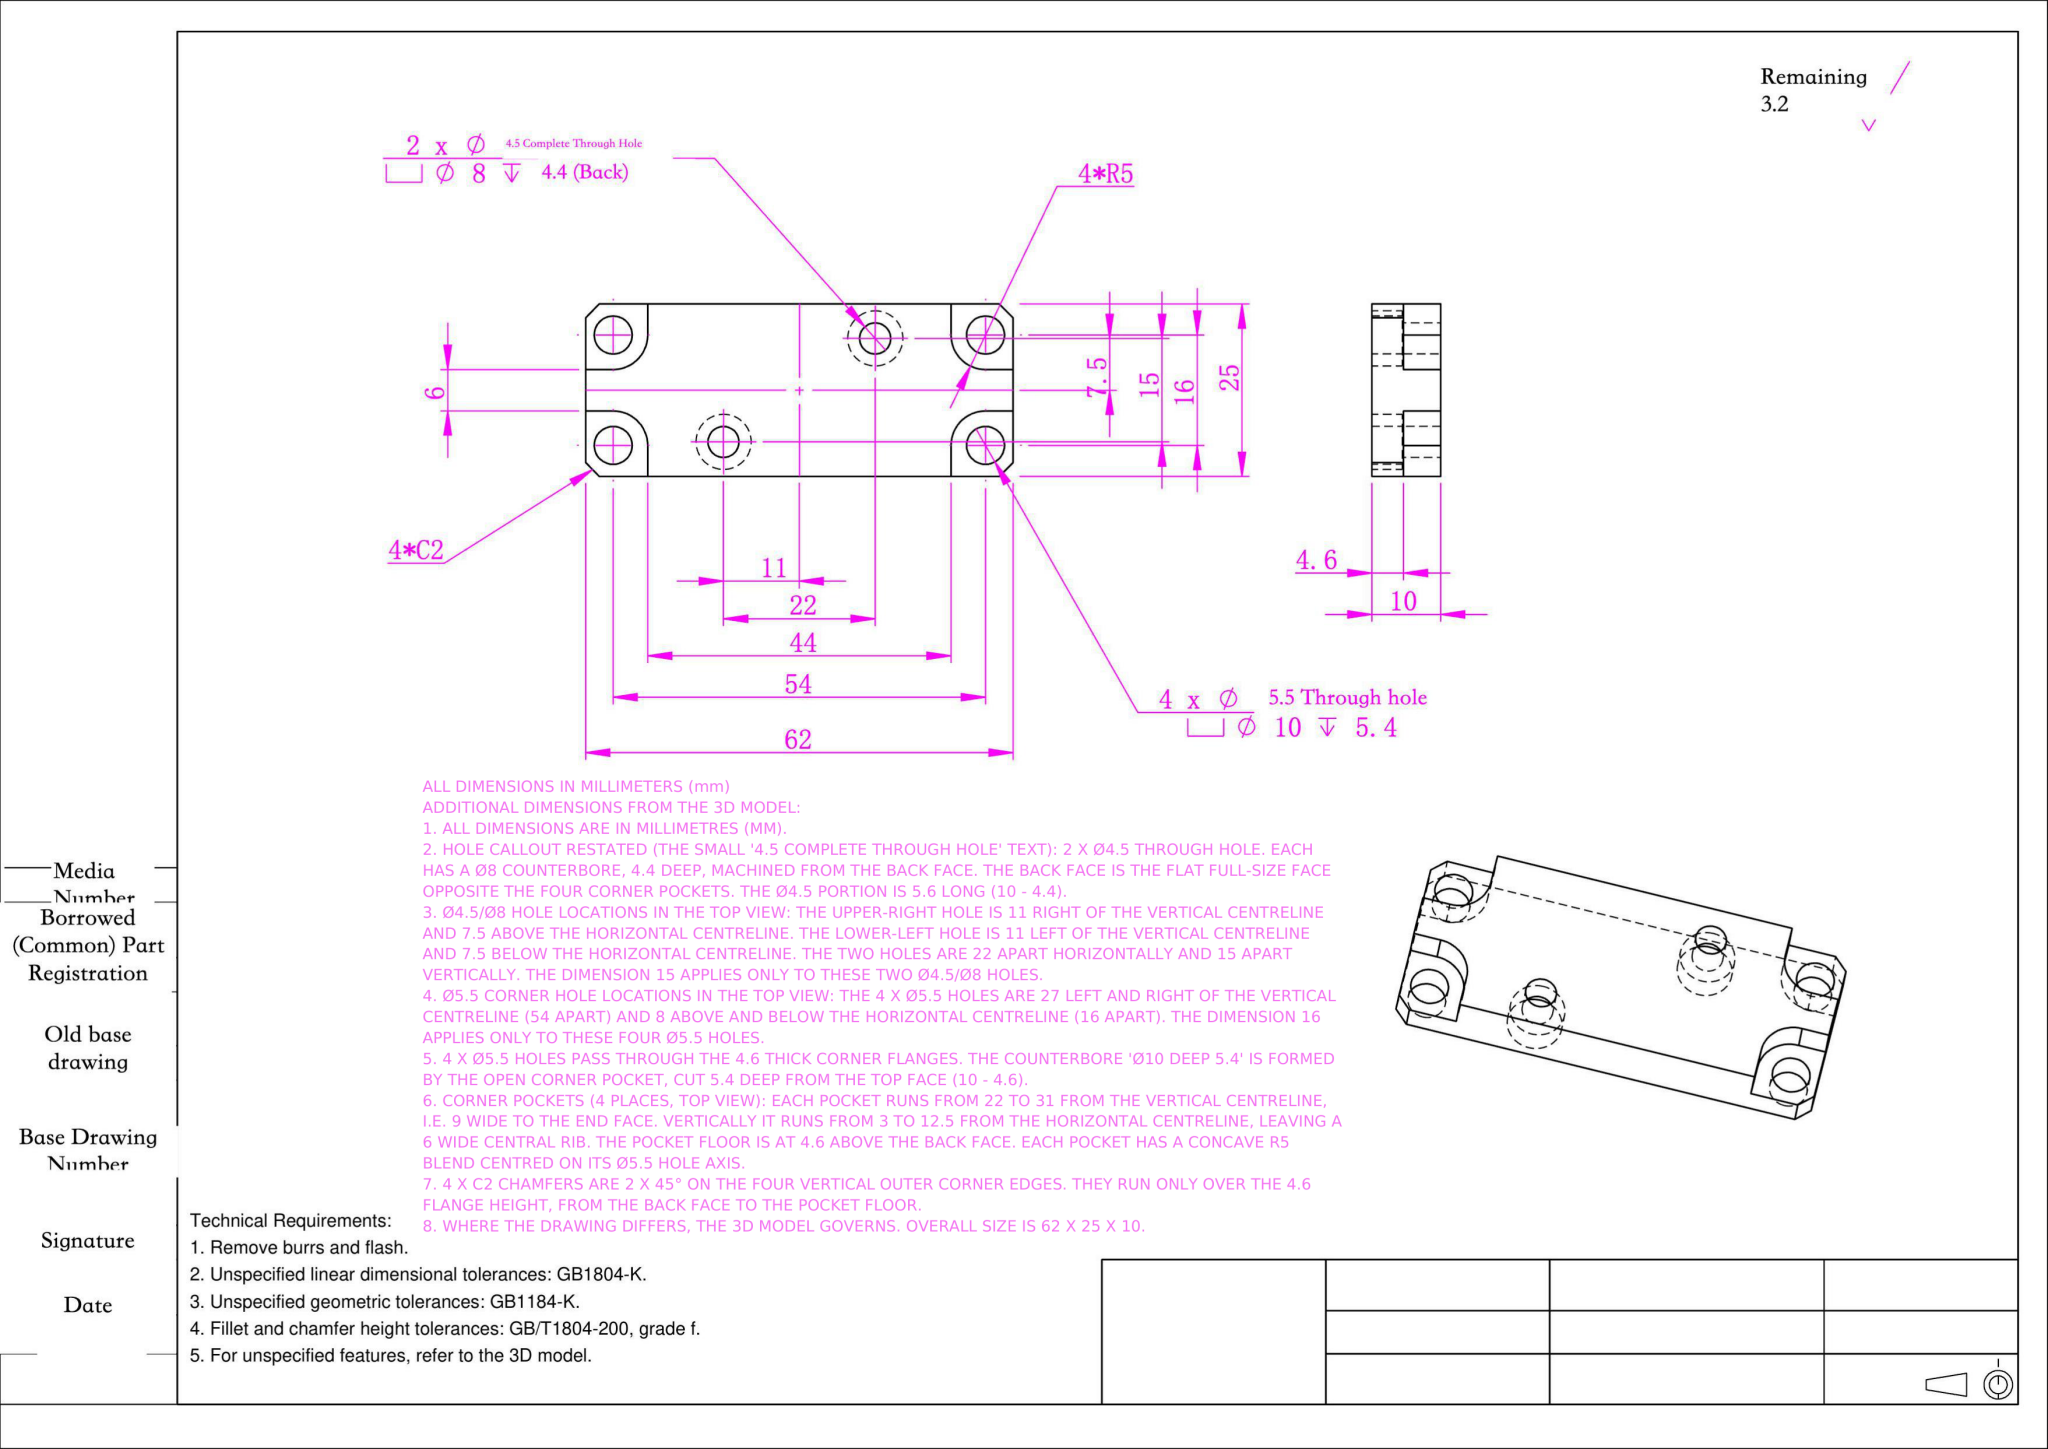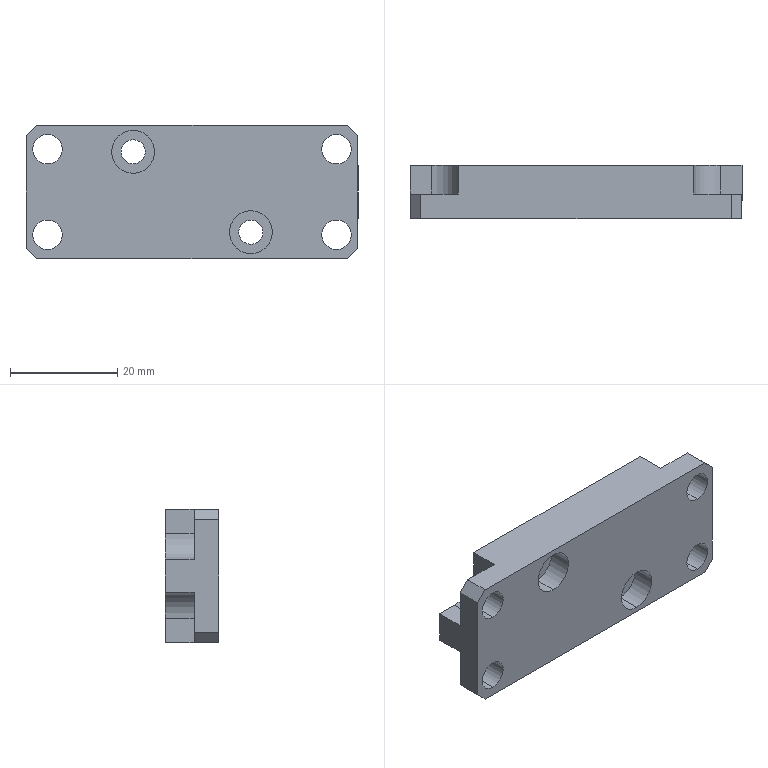Part | NX | mm | Notched Rail Bore Plate | 1 solid | 44 faces | box 62 x 10 x 25 mm | volume 12675 mm3 | plane 24 | cylinder 20 | commonest cylinder face diameters 5.5 x8 8 x4 4.5 x4 10 x4